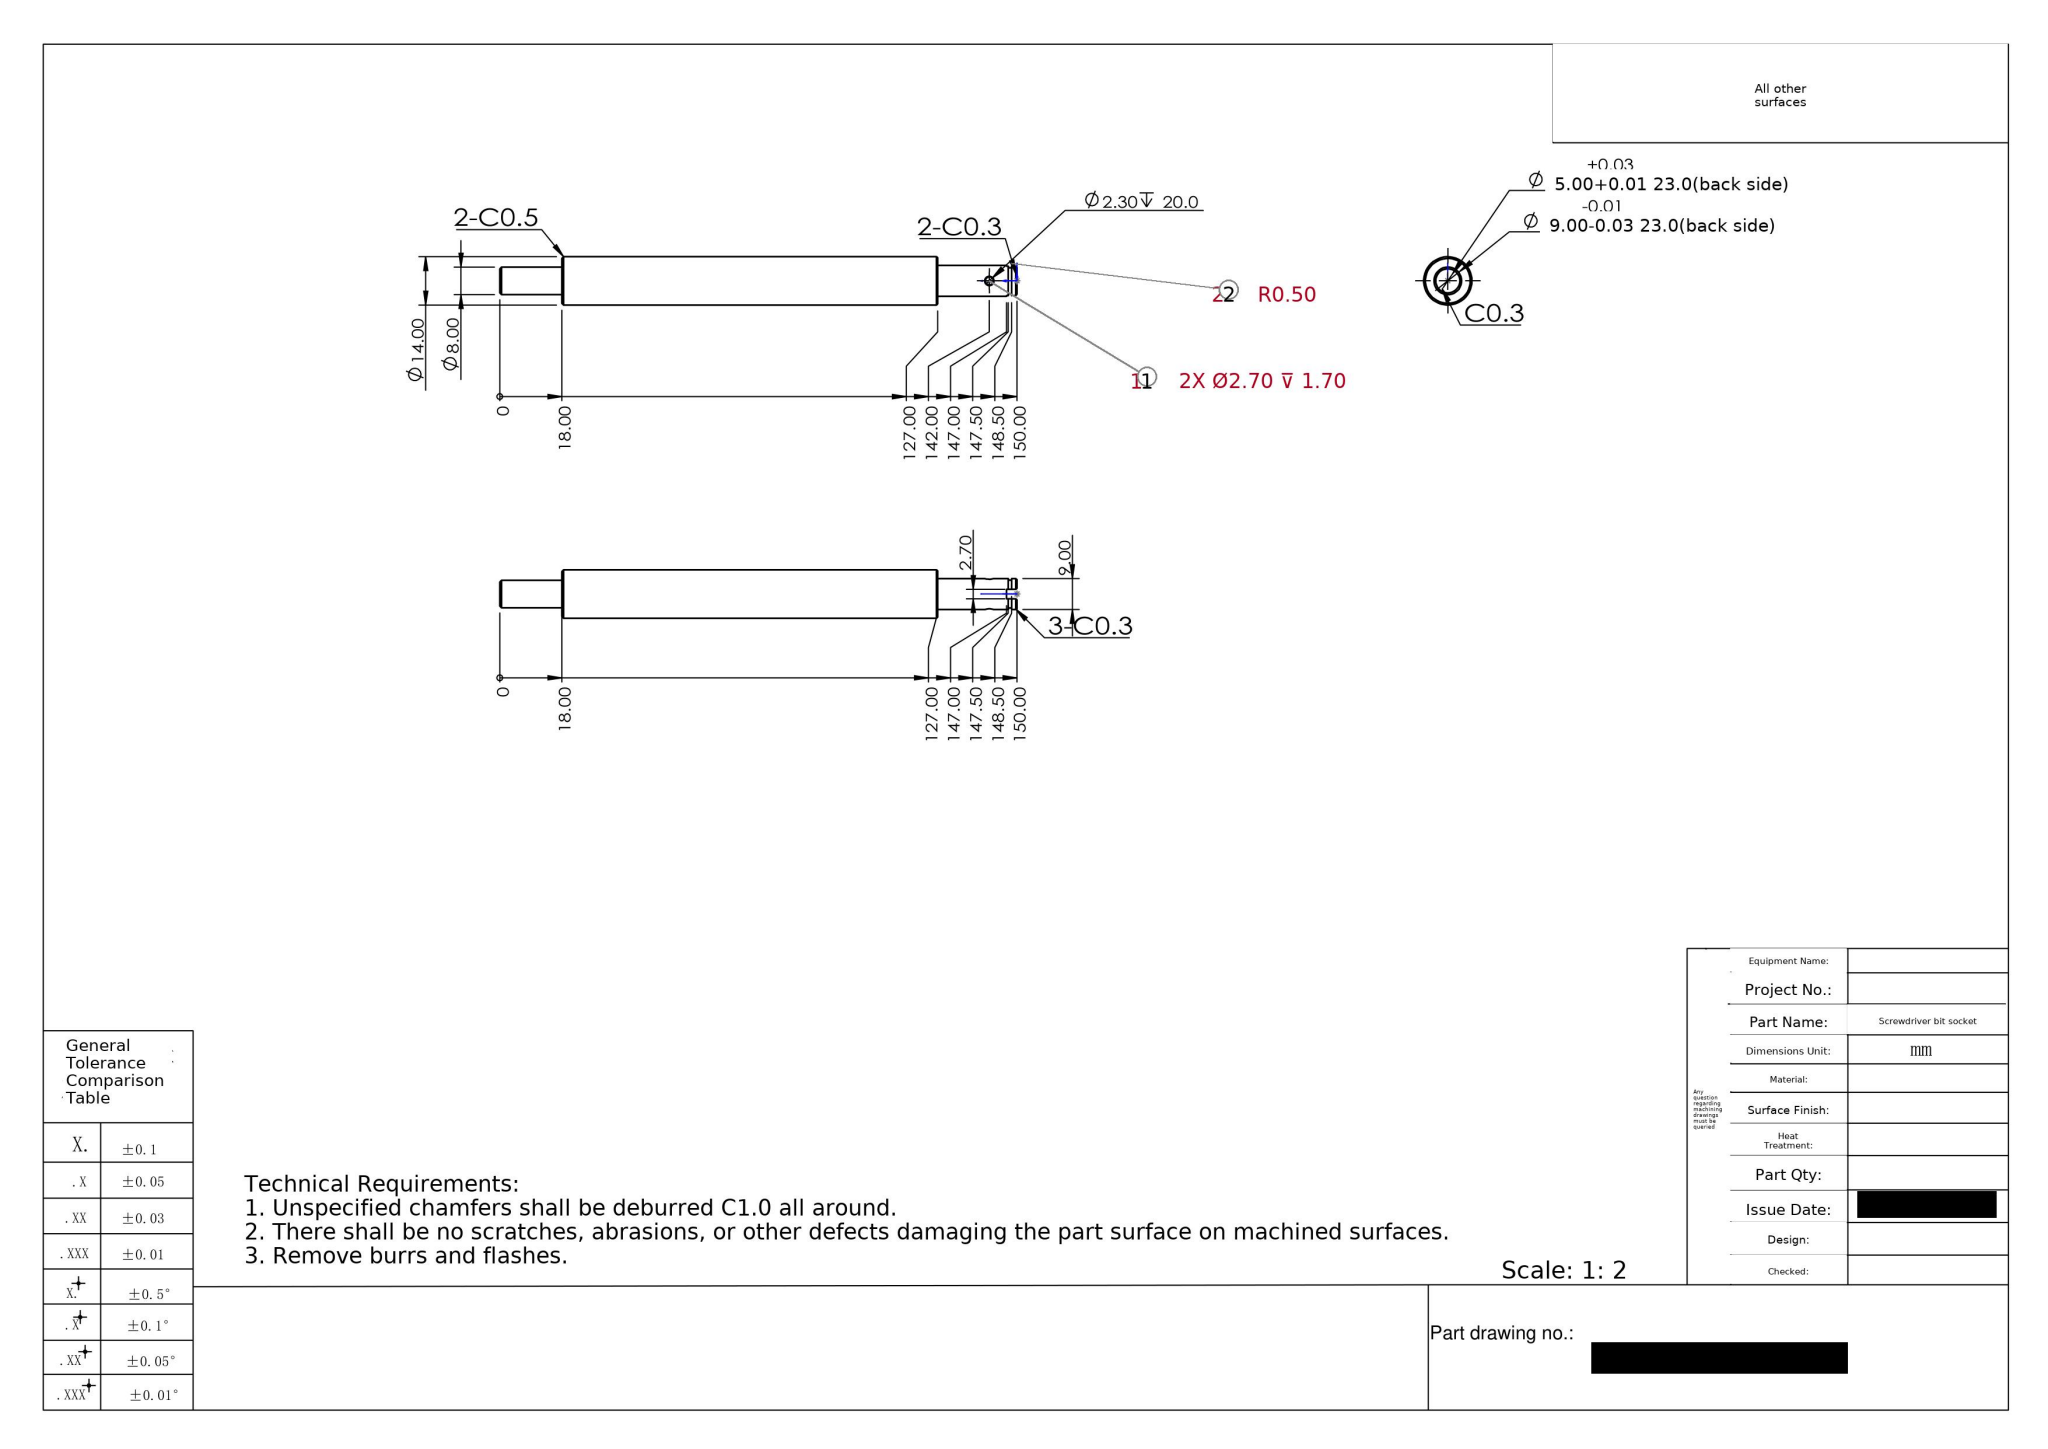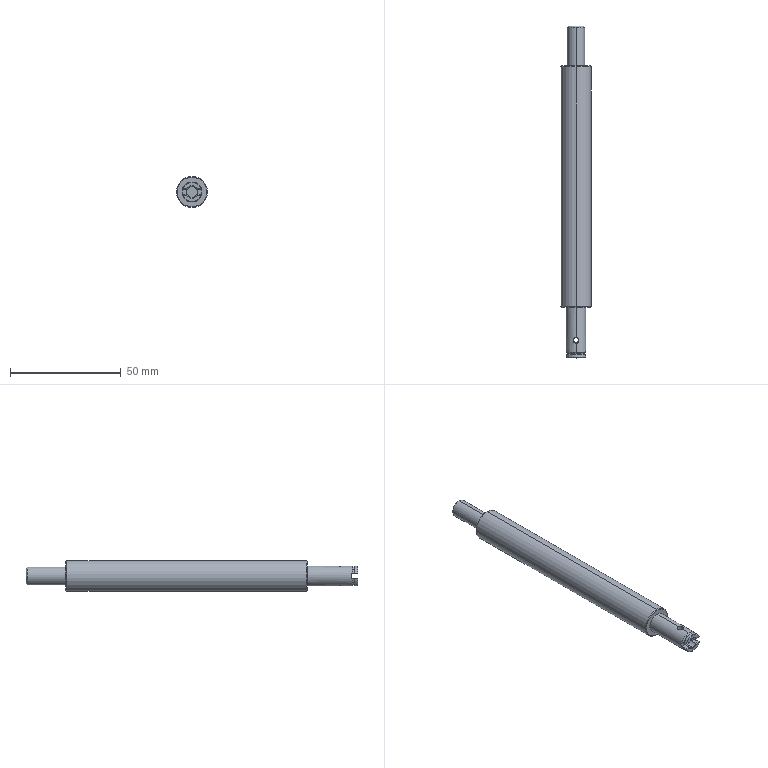Part | SolidWorks | mm | 1 solid | 55 faces | box 14 x 150 x 14 mm | volume 18620 mm3 | cylinder 19 | plane 18 | cone 12 | torus 6 | commonest cylinder face diameters 9 x5 2.7 x4 2.3 x4 5 x2 8 x2 14 x2
build123d program:
from build123d import *

# Parameters (mm, degrees)
SKETCH1_R           = 7
BOSS_EXTRUDE1_DEPTH = 132
SKETCH2_R           = 4
BOSS_EXTRUDE2_DEPTH = 18
CHAMFER1_SIZE       = 0.5
SKETCH3_W           = 14
SKETCH3_H           = 2.7
CUT_EXTRUDE1_DEPTH  = 3
SKETCH4_R           = 7
SKETCH4_R_2         = 4.5
SKETCH4_R_3         = 2.5
CUT_EXTRUDE2_DEPTH  = 23
SKETCH5_R           = 1.15
CUT_EXTRUDE3_DEPTH  = 10
CUT_EXTRUDE6_START  = -2.8
SKETCH7_R           = 1.35
CUT_EXTRUDE6_DEPTH  = 5
SKETCH6_R           = 0.5
CHAMFER2_SIZE       = 0.3


with BuildPart() as part:
    # Sketch1 → Boss-Extrude1 (new body)
    with BuildSketch(Plane(origin=(0, 0, 0), x_dir=(1, 0, 0), z_dir=(0, 1, 0))):
        with Locations(Location((0, 0, 0), (0, 0, 270))):
            Circle(SKETCH1_R)
    extrude(amount=BOSS_EXTRUDE1_DEPTH)

    # Sketch2 → Boss-Extrude2 (add)
    with BuildSketch(Plane(origin=(0, 132, 0), x_dir=(1, 0, 0), z_dir=(0, 1, 0))):
        with Locations(Location((0, 0, 0), (0, 0, 270))):
            Circle(SKETCH2_R)
    extrude(amount=BOSS_EXTRUDE2_DEPTH)

    # Chamfer1
    chamfer1_edges = [part.edges().sort_by_distance(p)[0] for p in [
        (0, 132, -7),
        (0, 150, -4),
    ]]
    chamfer(chamfer1_edges, length=CHAMFER1_SIZE)

    # Sketch3 → Cut-Extrude1 (cut)
    with BuildSketch(Plane.XZ):
        Rectangle(SKETCH3_W, SKETCH3_H)
    extrude(amount=-CUT_EXTRUDE1_DEPTH, mode=Mode.SUBTRACT)

    # Sketch4 → Cut-Extrude2 (cut)
    # profile 1 of 2: a face of its own
    with BuildSketch(Plane.XZ):
        with Locations(Location((0, 0, 0), (0, 0, 270))):
            Circle(SKETCH4_R)
        with Locations(Location((0, 0, 0), (0, 0, 270))):
            Circle(SKETCH4_R_2, mode=Mode.SUBTRACT)
    # profile 2 of 2: a face of its own
    with BuildSketch(Plane.XZ):
        with Locations(Location((0, 0, 0), (0, 0, 270))):
            Circle(SKETCH4_R_3)
    extrude(amount=-CUT_EXTRUDE2_DEPTH, mode=Mode.SUBTRACT)

    # Sketch5 → Cut-Extrude3 (cut, symmetric)
    with BuildSketch(Plane.XY):
        with Locations((0, 8)):
            Circle(SKETCH5_R)
    extrude(amount=CUT_EXTRUDE3_DEPTH, both=True, mode=Mode.SUBTRACT)

    # Sketch7 → Cut-Extrude6 (cut)
    with BuildSketch(Plane.XY.offset(CUT_EXTRUDE6_START)):
        with Locations((0, 8)):
            Circle(SKETCH7_R)
    cut_extrude6 = extrude(amount=-CUT_EXTRUDE6_DEPTH, mode=Mode.SUBTRACT)

    # Mirror1: Cut-Extrude6 across plane
    add(cut_extrude6.mirror(Plane.XY), mode=Mode.SUBTRACT)

    # Sketch6 → Cut-Revolve1 (revolve, cut)
    with BuildSketch(Plane(origin=(0, 0, 0), x_dir=(0, 0, -1), z_dir=(1, 0, 0))):
        with Locations((4.5, 2)):
            Circle(SKETCH6_R)
    revolve(axis=Axis((0, 0, 0), (0, 1, 0)), mode=Mode.SUBTRACT)

    # Chamfer2
    chamfer2_edges = [part.edges().sort_by_distance(p)[0] for p in [
        (-3.198, 0, -1.35),
        (3.198, 0, 1.35),
        (0, 0, 2.5),
        (1.199, 0, -2.194),
        (3.198, 0, -1.35),
        (-3.198, 0, 1.35),
        (0, 0, 4.5),
        (0, 0, -4.5),
        (0, 23, -7),
    ]]
    chamfer(chamfer2_edges, length=CHAMFER2_SIZE)


solid = part.part